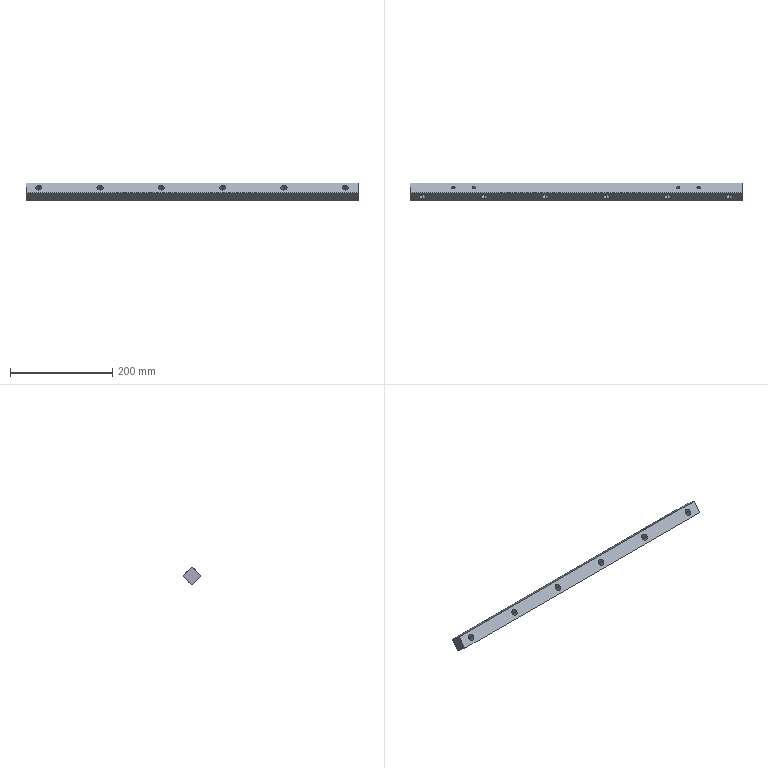Component | SolidWorks | OT-0100-001(HookSeat)-1 | 1 solid | 34 faces | box 650 x 35.17 x 35.17 mm | volume 384874 mm3 | cylinder 20 | cone 8 | plane 6 | commonest cylinder face diameters 12.5 x12 6.8 x8 | material Plain Carbon Steel
build123d program:
from build123d import *

# Parameters (mm, degrees)
SKETCH1_W             = 650
SKETCH1_H             = 25
BOSS_EXTRUDE1_DEPTH   = 25
CUT_EXTRUDE1_REACH    = 328.2
SKETCH2_R             = 6.25
M8_TAPPED_HOLE1_D     = 6.8
M8_TAPPED_HOLE1_DEPTH = 19.75
M8_TAPPED_HOLE1_TIP   = 2.043


with BuildPart() as part:
    # Sketch1 → Boss-Extrude1 (new body)
    with BuildSketch(Plane(origin=(0, 0, 0), x_dir=(1, 0, 0), z_dir=(0, 1, 0))):
        Rectangle(SKETCH1_W, SKETCH1_H)
    extrude(amount=BOSS_EXTRUDE1_DEPTH)

    # Sketch2 → Cut-Extrude1 (cut, up to next)
    with BuildSketch(Plane(origin=(0, 25, 0), x_dir=(1, 0, 0), z_dir=(0, 1, 0)), mode=Mode.PRIVATE) as cut_extrude1_sk1:
        with Locations(Location((300, 0, 0), (0, 0, 270))):
            Circle(SKETCH2_R)
    cut_extrude1_tool1 = extrude(cut_extrude1_sk1.sketch, amount=-CUT_EXTRUDE1_REACH, mode=Mode.PRIVATE) & part.part
    # Sketch2 → Cut-Extrude1 (cut, up to next)
    with BuildSketch(Plane(origin=(0, 25, 0), x_dir=(1, 0, 0), z_dir=(0, 1, 0)), mode=Mode.PRIVATE) as cut_extrude1_sk2:
        with Locations(Location((180, 0, 0), (0, 0, 270))):
            Circle(SKETCH2_R)
    cut_extrude1_tool2 = extrude(cut_extrude1_sk2.sketch, amount=-CUT_EXTRUDE1_REACH, mode=Mode.PRIVATE) & part.part
    # Sketch2 → Cut-Extrude1 (cut, up to next)
    with BuildSketch(Plane(origin=(0, 25, 0), x_dir=(1, 0, 0), z_dir=(0, 1, 0)), mode=Mode.PRIVATE) as cut_extrude1_sk3:
        with Locations(Location((60, 0, 0), (0, 0, 270))):
            Circle(SKETCH2_R)
    cut_extrude1_tool3 = extrude(cut_extrude1_sk3.sketch, amount=-CUT_EXTRUDE1_REACH, mode=Mode.PRIVATE) & part.part
    # Sketch2 → Cut-Extrude1 (cut, up to next)
    with BuildSketch(Plane(origin=(0, 25, 0), x_dir=(1, 0, 0), z_dir=(0, 1, 0)), mode=Mode.PRIVATE) as cut_extrude1_sk4:
        with Locations(Location((-60, 0, 0), (0, 0, 270))):
            Circle(SKETCH2_R)
    cut_extrude1_tool4 = extrude(cut_extrude1_sk4.sketch, amount=-CUT_EXTRUDE1_REACH, mode=Mode.PRIVATE) & part.part
    # Sketch2 → Cut-Extrude1 (cut, up to next)
    with BuildSketch(Plane(origin=(0, 25, 0), x_dir=(1, 0, 0), z_dir=(0, 1, 0)), mode=Mode.PRIVATE) as cut_extrude1_sk5:
        with Locations(Location((-180, 0, 0), (0, 0, 270))):
            Circle(SKETCH2_R)
    cut_extrude1_tool5 = extrude(cut_extrude1_sk5.sketch, amount=-CUT_EXTRUDE1_REACH, mode=Mode.PRIVATE) & part.part
    # Sketch2 → Cut-Extrude1 (cut, up to next)
    with BuildSketch(Plane(origin=(0, 25, 0), x_dir=(1, 0, 0), z_dir=(0, 1, 0)), mode=Mode.PRIVATE) as cut_extrude1_sk6:
        with Locations(Location((-300, 0, 0), (0, 0, 270))):
            Circle(SKETCH2_R)
    cut_extrude1_tool6 = extrude(cut_extrude1_sk6.sketch, amount=-CUT_EXTRUDE1_REACH, mode=Mode.PRIVATE) & part.part
    add(cut_extrude1_tool1.solids().sort_by_distance((300, 25, 0))[0], mode=Mode.SUBTRACT)
    add(cut_extrude1_tool2.solids().sort_by_distance((180, 25, 0))[0], mode=Mode.SUBTRACT)
    add(cut_extrude1_tool3.solids().sort_by_distance((60, 25, 0))[0], mode=Mode.SUBTRACT)
    add(cut_extrude1_tool4.solids().sort_by_distance((-60, 25, 0))[0], mode=Mode.SUBTRACT)
    add(cut_extrude1_tool5.solids().sort_by_distance((-180, 25, 0))[0], mode=Mode.SUBTRACT)
    add(cut_extrude1_tool6.solids().sort_by_distance((-300, 25, 0))[0], mode=Mode.SUBTRACT)

    # M8 Tapped Hole1
    with Locations(Plane.XY.offset(12.5)):
        with Locations((-240, 12.5), (240, 12.5), (-200, 12.5), (200, 12.5)):
            Hole(M8_TAPPED_HOLE1_D / 2, depth=M8_TAPPED_HOLE1_DEPTH)
            with Locations((0, 0, -(M8_TAPPED_HOLE1_DEPTH + M8_TAPPED_HOLE1_TIP / 2))):  # 118° drill point
                Cone(0, M8_TAPPED_HOLE1_D / 2, M8_TAPPED_HOLE1_TIP, mode=Mode.SUBTRACT)


solid = part.part

# Placed as in the assembly
solid = solid.moved(Location((200, -106.658, 142.812), (-39.097, 0, 0)))
STEP:
#1=COLOUR_RGB('',0.7922,0.8196,0.9333);
#2=FILL_AREA_STYLE_COLOUR('',#1);
#3=FILL_AREA_STYLE('',(#2));
#4=SURFACE_STYLE_FILL_AREA(#3);
#5=SURFACE_SIDE_STYLE('',(#4));
#6=SURFACE_STYLE_USAGE(.BOTH.,#5);
#7=PRESENTATION_STYLE_ASSIGNMENT((#6));
#8=CARTESIAN_POINT('',(-1.709,-3.997,5.091));
#9=VERTEX_POINT('',#8);
#10=CARTESIAN_POINT('',(-1.441,-3.997,5.091));
#11=VERTEX_POINT('',#10);
#12=CARTESIAN_POINT('',(-1.575,-3.997,5.091));
#13=DIRECTION('',(0.,0.6306,0.7761));
#14=DIRECTION('',(1.,0.,0.));
#15=AXIS2_PLACEMENT_3D('',#12,#13,#14);
#16=CIRCLE('',#15,0.1339);
#17=EDGE_CURVE('',#9,#11,#16,.T.);
#18=ORIENTED_EDGE('',*,*,#17,.F.);
#19=CARTESIAN_POINT('',(-1.709,-3.507,5.694));
#20=VERTEX_POINT('',#19);
#21=CARTESIAN_POINT('',(-1.709,-3.507,5.694));
#22=DIRECTION('',(0.,0.6306,0.7761));
#23=VECTOR('',#22,39.37);
#24=LINE('',#21,#23);
#25=EDGE_CURVE('',#9,#20,#24,.T.);
#26=ORIENTED_EDGE('',*,*,#25,.T.);
#27=CARTESIAN_POINT('',(-1.441,-3.507,5.694));
#28=VERTEX_POINT('',#27);
#29=CARTESIAN_POINT('',(-1.575,-3.507,5.694));
#30=DIRECTION('',(0.,0.6306,0.7761));
#31=DIRECTION('',(1.,0.,0.));
#32=AXIS2_PLACEMENT_3D('',#29,#30,#31);
#33=CIRCLE('',#32,0.1339);
#34=EDGE_CURVE('',#20,#28,#33,.T.);
#35=ORIENTED_EDGE('',*,*,#34,.T.);
#36=CARTESIAN_POINT('',(-1.441,-3.507,5.694));
#37=DIRECTION('',(0.,0.6306,0.7761));
#38=VECTOR('',#37,39.37);
#39=LINE('',#36,#38);
#40=EDGE_CURVE('',#11,#28,#39,.T.);
#41=ORIENTED_EDGE('',*,*,#40,.F.);
#42=EDGE_LOOP('',(#18,#26,#35,#41));
#43=FACE_OUTER_BOUND('',#42,.T.);
#44=CARTESIAN_POINT('',(-1.575,-3.507,5.694));
#45=DIRECTION('',(0.,0.6306,0.7761));
#46=DIRECTION('',(1.,0.,0.));
#47=AXIS2_PLACEMENT_3D('',#44,#45,#46);
#48=CYLINDRICAL_SURFACE('',#47,0.1339);
#49=ADVANCED_FACE('',(#43),#48,.F.);
#50=CARTESIAN_POINT('',(-1.575,-4.048,5.028));
#51=VERTEX_POINT('',#50);
#52=CARTESIAN_POINT('',(-1.441,-3.997,5.091));
#53=DIRECTION('',(0.8572,0.3248,0.3997));
#54=VECTOR('',#53,39.37);
#55=LINE('',#52,#54);
#56=EDGE_CURVE('',#51,#11,#55,.T.);
#57=ORIENTED_EDGE('',*,*,#56,.F.);
#58=CARTESIAN_POINT('',(-1.709,-3.997,5.091));
#59=DIRECTION('',(-0.8572,0.3248,0.3997));
#60=VECTOR('',#59,39.37);
#61=LINE('',#58,#60);
#62=EDGE_CURVE('',#51,#9,#61,.T.);
#63=ORIENTED_EDGE('',*,*,#62,.T.);
#64=ORIENTED_EDGE('',*,*,#17,.T.);
#65=EDGE_LOOP('',(#57,#63,#64));
#66=FACE_OUTER_BOUND('',#65,.T.);
#67=CARTESIAN_POINT('',(-1.575,-3.997,5.091));
#68=DIRECTION('',(0.,0.6306,0.7761));
#69=DIRECTION('',(1.,0.,0.));
#70=AXIS2_PLACEMENT_3D('',#67,#68,#69);
#71=CONICAL_SURFACE('',#70,0.1339,1.03);
#72=ADVANCED_FACE('',(#66),#71,.F.);
#73=CARTESIAN_POINT('',(17.189,-3.997,5.091));
#74=VERTEX_POINT('',#73);
#75=CARTESIAN_POINT('',(17.457,-3.997,5.091));
#76=VERTEX_POINT('',#75);
#77=CARTESIAN_POINT('',(17.323,-3.997,5.091));
#78=DIRECTION('',(0.,0.6306,0.7761));
#79=DIRECTION('',(1.,0.,0.));
#80=AXIS2_PLACEMENT_3D('',#77,#78,#79);
#81=CIRCLE('',#80,0.1339);
#82=EDGE_CURVE('',#74,#76,#81,.T.);
#83=ORIENTED_EDGE('',*,*,#82,.F.);
#84=CARTESIAN_POINT('',(17.189,-3.507,5.694));
#85=VERTEX_POINT('',#84);
#86=CARTESIAN_POINT('',(17.189,-3.507,5.694));
#87=DIRECTION('',(0.,0.6306,0.7761));
#88=VECTOR('',#87,39.37);
#89=LINE('',#86,#88);
#90=EDGE_CURVE('',#74,#85,#89,.T.);
#91=ORIENTED_EDGE('',*,*,#90,.T.);
#92=CARTESIAN_POINT('',(17.457,-3.507,5.694));
#93=VERTEX_POINT('',#92);
#94=CARTESIAN_POINT('',(17.323,-3.507,5.694));
#95=DIRECTION('',(0.,0.6306,0.7761));
#96=DIRECTION('',(1.,0.,0.));
#97=AXIS2_PLACEMENT_3D('',#94,#95,#96);
#98=CIRCLE('',#97,0.1339);
#99=EDGE_CURVE('',#85,#93,#98,.T.);
#100=ORIENTED_EDGE('',*,*,#99,.T.);
#101=CARTESIAN_POINT('',(17.457,-3.507,5.694));
#102=DIRECTION('',(0.,0.6306,0.7761));
#103=VECTOR('',#102,39.37);
#104=LINE('',#101,#103);
#105=EDGE_CURVE('',#76,#93,#104,.T.);
#106=ORIENTED_EDGE('',*,*,#105,.F.);
#107=EDGE_LOOP('',(#83,#91,#100,#106));
#108=FACE_OUTER_BOUND('',#107,.T.);
#109=CARTESIAN_POINT('',(17.323,-3.507,5.694));
#110=DIRECTION('',(0.,0.6306,0.7761));
#111=DIRECTION('',(1.,0.,0.));
#112=AXIS2_PLACEMENT_3D('',#109,#110,#111);
#113=CYLINDRICAL_SURFACE('',#112,0.1339);
#114=ADVANCED_FACE('',(#108),#113,.F.);
#115=CARTESIAN_POINT('',(17.323,-4.048,5.028));
#116=VERTEX_POINT('',#115);
#117=CARTESIAN_POINT('',(17.457,-3.997,5.091));
#118=DIRECTION('',(0.8572,0.3248,0.3997));
#119=VECTOR('',#118,39.37);
#120=LINE('',#117,#119);
#121=EDGE_CURVE('',#116,#76,#120,.T.);
#122=ORIENTED_EDGE('',*,*,#121,.F.);
#123=CARTESIAN_POINT('',(17.189,-3.997,5.091));
#124=DIRECTION('',(-0.8572,0.3248,0.3997));
#125=VECTOR('',#124,39.37);
#126=LINE('',#123,#125);
#127=EDGE_CURVE('',#116,#74,#126,.T.);
#128=ORIENTED_EDGE('',*,*,#127,.T.);
#129=ORIENTED_EDGE('',*,*,#82,.T.);
#130=EDGE_LOOP('',(#122,#128,#129));
#131=FACE_OUTER_BOUND('',#130,.T.);
#132=CARTESIAN_POINT('',(17.323,-3.997,5.091));
#133=DIRECTION('',(0.,0.6306,0.7761));
#134=DIRECTION('',(1.,0.,0.));
#135=AXIS2_PLACEMENT_3D('',#132,#133,#134);
#136=CONICAL_SURFACE('',#135,0.1339,1.03);
#137=ADVANCED_FACE('',(#131),#136,.F.);
#138=CARTESIAN_POINT('',(-0.1339,-3.997,5.091));
#139=VERTEX_POINT('',#138);
#140=CARTESIAN_POINT('',(0.1339,-3.997,5.091));
#141=VERTEX_POINT('',#140);
#142=CARTESIAN_POINT('',(0.,-3.997,5.091));
#143=DIRECTION('',(0.,0.6306,0.7761));
#144=DIRECTION('',(1.,0.,0.));
#145=AXIS2_PLACEMENT_3D('',#142,#143,#144);
#146=CIRCLE('',#145,0.1339);
#147=EDGE_CURVE('',#139,#141,#146,.T.);
#148=ORIENTED_EDGE('',*,*,#147,.F.);
#149=CARTESIAN_POINT('',(-0.1339,-3.507,5.694));
#150=VERTEX_POINT('',#149);
#151=CARTESIAN_POINT('',(-0.1339,-3.507,5.694));
#152=DIRECTION('',(0.,0.6306,0.7761));
#153=VECTOR('',#152,39.37);
#154=LINE('',#151,#153);
#155=EDGE_CURVE('',#139,#150,#154,.T.);
#156=ORIENTED_EDGE('',*,*,#155,.T.);
#157=CARTESIAN_POINT('',(0.1339,-3.507,5.694));
#158=VERTEX_POINT('',#157);
#159=CARTESIAN_POINT('',(0.,-3.507,5.694));
#160=DIRECTION('',(0.,0.6306,0.7761));
#161=DIRECTION('',(1.,0.,0.));
#162=AXIS2_PLACEMENT_3D('',#159,#160,#161);
#163=CIRCLE('',#162,0.1339);
#164=EDGE_CURVE('',#150,#158,#163,.T.);
#165=ORIENTED_EDGE('',*,*,#164,.T.);
#166=CARTESIAN_POINT('',(0.1339,-3.507,5.694));
#167=DIRECTION('',(0.,0.6306,0.7761));
#168=VECTOR('',#167,39.37);
#169=LINE('',#166,#168);
#170=EDGE_CURVE('',#141,#158,#169,.T.);
#171=ORIENTED_EDGE('',*,*,#170,.F.);
#172=EDGE_LOOP('',(#148,#156,#165,#171));
#173=FACE_OUTER_BOUND('',#172,.T.);
#174=CARTESIAN_POINT('',(0.,-3.507,5.694));
#175=DIRECTION('',(0.,0.6306,0.7761));
#176=DIRECTION('',(1.,0.,0.));
#177=AXIS2_PLACEMENT_3D('',#174,#175,#176);
#178=CYLINDRICAL_SURFACE('',#177,0.1339);
#179=ADVANCED_FACE('',(#173),#178,.F.);
#180=CARTESIAN_POINT('',(0.,-4.048,5.028));
#181=VERTEX_POINT('',#180);
#182=CARTESIAN_POINT('',(0.1339,-3.997,5.091));
#183=DIRECTION('',(0.8572,0.3248,0.3997));
#184=VECTOR('',#183,39.37);
#185=LINE('',#182,#184);
#186=EDGE_CURVE('',#181,#141,#185,.T.);
#187=ORIENTED_EDGE('',*,*,#186,.F.);
#188=CARTESIAN_POINT('',(-0.1339,-3.997,5.091));
#189=DIRECTION('',(-0.8572,0.3248,0.3997));
#190=VECTOR('',#189,39.37);
#191=LINE('',#188,#190);
#192=EDGE_CURVE('',#181,#139,#191,.T.);
#193=ORIENTED_EDGE('',*,*,#192,.T.);
#194=ORIENTED_EDGE('',*,*,#147,.T.);
#195=EDGE_LOOP('',(#187,#193,#194));
#196=FACE_OUTER_BOUND('',#195,.T.);
#197=CARTESIAN_POINT('',(0.,-3.997,5.091));
#198=DIRECTION('',(0.,0.6306,0.7761));
#199=DIRECTION('',(1.,0.,0.));
#200=AXIS2_PLACEMENT_3D('',#197,#198,#199);
#201=CONICAL_SURFACE('',#200,0.1339,1.03);
#202=ADVANCED_FACE('',(#196),#201,.F.);
#203=CARTESIAN_POINT('',(15.614,-3.997,5.091));
#204=VERTEX_POINT('',#203);
#205=CARTESIAN_POINT('',(15.882,-3.997,5.091));
#206=VERTEX_POINT('',#205);
#207=CARTESIAN_POINT('',(15.748,-3.997,5.091));
#208=DIRECTION('',(0.,0.6306,0.7761));
#209=DIRECTION('',(1.,0.,0.));
#210=AXIS2_PLACEMENT_3D('',#207,#208,#209);
#211=CIRCLE('',#210,0.1339);
#212=EDGE_CURVE('',#204,#206,#211,.T.);
#213=ORIENTED_EDGE('',*,*,#212,.F.);
#214=CARTESIAN_POINT('',(15.614,-3.507,5.694));
#215=VERTEX_POINT('',#214);
#216=CARTESIAN_POINT('',(15.614,-3.507,5.694));
#217=DIRECTION('',(0.,0.6306,0.7761));
#218=VECTOR('',#217,39.37);
#219=LINE('',#216,#218);
#220=EDGE_CURVE('',#204,#215,#219,.T.);
#221=ORIENTED_EDGE('',*,*,#220,.T.);
#222=CARTESIAN_POINT('',(15.882,-3.507,5.694));
#223=VERTEX_POINT('',#222);
#224=CARTESIAN_POINT('',(15.748,-3.507,5.694));
#225=DIRECTION('',(0.,0.6306,0.7761));
#226=DIRECTION('',(1.,0.,0.));
#227=AXIS2_PLACEMENT_3D('',#224,#225,#226);
#228=CIRCLE('',#227,0.1339);
#229=EDGE_CURVE('',#215,#223,#228,.T.);
#230=ORIENTED_EDGE('',*,*,#229,.T.);
#231=CARTESIAN_POINT('',(15.882,-3.507,5.694));
#232=DIRECTION('',(0.,0.6306,0.7761));
#233=VECTOR('',#232,39.37);
#234=LINE('',#231,#233);
#235=EDGE_CURVE('',#206,#223,#234,.T.);
#236=ORIENTED_EDGE('',*,*,#235,.F.);
#237=EDGE_LOOP('',(#213,#221,#230,#236));
#238=FACE_OUTER_BOUND('',#237,.T.);
#239=CARTESIAN_POINT('',(15.748,-3.507,5.694));
#240=DIRECTION('',(0.,0.6306,0.7761));
#241=DIRECTION('',(1.,0.,0.));
#242=AXIS2_PLACEMENT_3D('',#239,#240,#241);
#243=CYLINDRICAL_SURFACE('',#242,0.1339);
#244=ADVANCED_FACE('',(#238),#243,.F.);
#245=CARTESIAN_POINT('',(15.748,-4.048,5.028));
#246=VERTEX_POINT('',#245);
#247=CARTESIAN_POINT('',(15.882,-3.997,5.091));
#248=DIRECTION('',(0.8572,0.3248,0.3997));
#249=VECTOR('',#248,39.37);
#250=LINE('',#247,#249);
#251=EDGE_CURVE('',#246,#206,#250,.T.);
#252=ORIENTED_EDGE('',*,*,#251,.F.);
#253=CARTESIAN_POINT('',(15.614,-3.997,5.091));
#254=DIRECTION('',(-0.8572,0.3248,0.3997));
#255=VECTOR('',#254,39.37);
#256=LINE('',#253,#255);
#257=EDGE_CURVE('',#246,#204,#256,.T.);
#258=ORIENTED_EDGE('',*,*,#257,.T.);
#259=ORIENTED_EDGE('',*,*,#212,.T.);
#260=EDGE_LOOP('',(#252,#258,#259));
#261=FACE_OUTER_BOUND('',#260,.T.);
#262=CARTESIAN_POINT('',(15.748,-3.997,5.091));
#263=DIRECTION('',(0.,0.6306,0.7761));
#264=DIRECTION('',(1.,0.,0.));
#265=AXIS2_PLACEMENT_3D('',#262,#263,#264);
#266=CONICAL_SURFACE('',#265,0.1339,1.03);
#267=ADVANCED_FACE('',(#261),#266,.F.);
#268=CARTESIAN_POINT('',(-3.937,-4.354,5.432));
#269=VERTEX_POINT('',#268);
#270=CARTESIAN_POINT('',(-3.937,-4.044,5.813));
#271=VERTEX_POINT('',#270);
#272=CARTESIAN_POINT('',(-3.937,-4.199,5.623));
#273=DIRECTION('',(-0.,0.7761,-0.6306));
#274=DIRECTION('',(0.,-0.6306,-0.7761));
#275=AXIS2_PLACEMENT_3D('',#272,#273,#274);
#276=CIRCLE('',#275,0.2461);
#277=EDGE_CURVE('',#269,#271,#276,.T.);
#278=ORIENTED_EDGE('',*,*,#277,.F.);
#279=CARTESIAN_POINT('',(-3.937,-3.59,4.811));
#280=VERTEX_POINT('',#279);
#281=CARTESIAN_POINT('',(-3.937,-4.354,5.432));
#282=DIRECTION('',(-0.,0.7761,-0.6306));
#283=VECTOR('',#282,39.37);
#284=LINE('',#281,#283);
#285=EDGE_CURVE('',#269,#280,#284,.T.);
#286=ORIENTED_EDGE('',*,*,#285,.T.);
#287=CARTESIAN_POINT('',(-3.937,-3.28,5.193));
#288=VERTEX_POINT('',#287);
#289=CARTESIAN_POINT('',(-3.937,-3.435,5.002));
#290=DIRECTION('',(-0.,0.7761,-0.6306));
#291=DIRECTION('',(0.,0.6306,0.7761));
#292=AXIS2_PLACEMENT_3D('',#289,#290,#291);
#293=CIRCLE('',#292,0.2461);
#294=EDGE_CURVE('',#280,#288,#293,.T.);
#295=ORIENTED_EDGE('',*,*,#294,.T.);
#296=CARTESIAN_POINT('',(-3.937,-4.044,5.814));
#297=DIRECTION('',(-0.,0.7761,-0.6306));
#298=VECTOR('',#297,39.37);
#299=LINE('',#296,#298);
#300=EDGE_CURVE('',#271,#288,#299,.T.);
#301=ORIENTED_EDGE('',*,*,#300,.F.);
#302=EDGE_LOOP('',(#278,#286,#295,#301));
#303=FACE_OUTER_BOUND('',#302,.T.);
#304=CARTESIAN_POINT('',(-3.937,-4.199,5.623));
#305=DIRECTION('',(-0.,0.7761,-0.6306));
#306=DIRECTION('',(0.,0.6306,0.7761));
#307=AXIS2_PLACEMENT_3D('',#304,#305,#306);
#308=CYLINDRICAL_SURFACE('',#307,0.2461);
#309=ADVANCED_FACE('',(#303),#308,.F.);
#310=CARTESIAN_POINT('',(0.7874,-4.354,5.432));
#311=VERTEX_POINT('',#310);
#312=CARTESIAN_POINT('',(0.7874,-4.044,5.813));
#313=VERTEX_POINT('',#312);
#314=CARTESIAN_POINT('',(0.7874,-4.199,5.623));
#315=DIRECTION('',(-0.,0.7761,-0.6306));
#316=DIRECTION('',(0.,-0.6306,-0.7761));
#317=AXIS2_PLACEMENT_3D('',#314,#315,#316);
#318=CIRCLE('',#317,0.2461);
#319=EDGE_CURVE('',#311,#313,#318,.T.);
#320=ORIENTED_EDGE('',*,*,#319,.F.);
#321=CARTESIAN_POINT('',(0.7874,-3.59,4.811));
#322=VERTEX_POINT('',#321);
#323=CARTESIAN_POINT('',(0.7874,-4.354,5.432));
#324=DIRECTION('',(-0.,0.7761,-0.6306));
#325=VECTOR('',#324,39.37);
#326=LINE('',#323,#325);
#327=EDGE_CURVE('',#311,#322,#326,.T.);
#328=ORIENTED_EDGE('',*,*,#327,.T.);
#329=CARTESIAN_POINT('',(0.7874,-3.28,5.193));
#330=VERTEX_POINT('',#329);
#331=CARTESIAN_POINT('',(0.7874,-3.435,5.002));
#332=DIRECTION('',(-0.,0.7761,-0.6306));
#333=DIRECTION('',(0.,0.6306,0.7761));
#334=AXIS2_PLACEMENT_3D('',#331,#332,#333);
#335=CIRCLE('',#334,0.2461);
#336=EDGE_CURVE('',#322,#330,#335,.T.);
#337=ORIENTED_EDGE('',*,*,#336,.T.);
#338=CARTESIAN_POINT('',(0.7874,-4.044,5.814));
#339=DIRECTION('',(-0.,0.7761,-0.6306));
#340=VECTOR('',#339,39.37);
#341=LINE('',#338,#340);
#342=EDGE_CURVE('',#313,#330,#341,.T.);
#343=ORIENTED_EDGE('',*,*,#342,.F.);
#344=EDGE_LOOP('',(#320,#328,#337,#343));
#345=FACE_OUTER_BOUND('',#344,.T.);
#346=CARTESIAN_POINT('',(0.7874,-4.199,5.623));
#347=DIRECTION('',(-0.,0.7761,-0.6306));
#348=DIRECTION('',(0.,0.6306,0.7761));
#349=AXIS2_PLACEMENT_3D('',#346,#347,#348);
#350=CYLINDRICAL_SURFACE('',#349,0.2461);
#351=ADVANCED_FACE('',(#345),#350,.F.);
#352=CARTESIAN_POINT('',(5.512,-4.354,5.432));
#353=VERTEX_POINT('',#352);
#354=CARTESIAN_POINT('',(5.512,-4.044,5.813));
#355=VERTEX_POINT('',#354);
#356=CARTESIAN_POINT('',(5.512,-4.199,5.623));
#357=DIRECTION('',(-0.,0.7761,-0.6306));
#358=DIRECTION('',(0.,-0.6306,-0.7761));
#359=AXIS2_PLACEMENT_3D('',#356,#357,#358);
#360=CIRCLE('',#359,0.2461);
#361=EDGE_CURVE('',#353,#355,#360,.T.);
#362=ORIENTED_EDGE('',*,*,#361,.F.);
#363=CARTESIAN_POINT('',(5.512,-3.59,4.811));
#364=VERTEX_POINT('',#363);
#365=CARTESIAN_POINT('',(5.512,-4.354,5.432));
#366=DIRECTION('',(-0.,0.7761,-0.6306));
#367=VECTOR('',#366,39.37);
#368=LINE('',#365,#367);
#369=EDGE_CURVE('',#353,#364,#368,.T.);
#370=ORIENTED_EDGE('',*,*,#369,.T.);
#371=CARTESIAN_POINT('',(5.512,-3.28,5.193));
#372=VERTEX_POINT('',#371);
#373=CARTESIAN_POINT('',(5.512,-3.435,5.002));
#374=DIRECTION('',(-0.,0.7761,-0.6306));
#375=DIRECTION('',(0.,0.6306,0.7761));
#376=AXIS2_PLACEMENT_3D('',#373,#374,#375);
#377=CIRCLE('',#376,0.2461);
#378=EDGE_CURVE('',#364,#372,#377,.T.);
#379=ORIENTED_EDGE('',*,*,#378,.T.);
#380=CARTESIAN_POINT('',(5.512,-4.044,5.814));
#381=DIRECTION('',(-0.,0.7761,-0.6306));
#382=VECTOR('',#381,39.37);
#383=LINE('',#380,#382);
#384=EDGE_CURVE('',#355,#372,#383,.T.);
#385=ORIENTED_EDGE('',*,*,#384,.F.);
#386=EDGE_LOOP('',(#362,#370,#379,#385));
#387=FACE_OUTER_BOUND('',#386,.T.);
#388=CARTESIAN_POINT('',(5.512,-4.199,5.623));
#389=DIRECTION('',(-0.,0.7761,-0.6306));
#390=DIRECTION('',(0.,0.6306,0.7761));
#391=AXIS2_PLACEMENT_3D('',#388,#389,#390);
#392=CYLINDRICAL_SURFACE('',#391,0.2461);
#393=ADVANCED_FACE('',(#387),#392,.F.);
#394=CARTESIAN_POINT('',(10.236,-4.354,5.432));
#395=VERTEX_POINT('',#394);
#396=CARTESIAN_POINT('',(10.236,-4.044,5.813));
#397=VERTEX_POINT('',#396);
#398=CARTESIAN_POINT('',(10.236,-4.199,5.623));
#399=DIRECTION('',(-0.,0.7761,-0.6306));
#400=DIRECTION('',(0.,-0.6306,-0.7761));
#401=AXIS2_PLACEMENT_3D('',#398,#399,#400);
#402=CIRCLE('',#401,0.2461);
#403=EDGE_CURVE('',#395,#397,#402,.T.);
#404=ORIENTED_EDGE('',*,*,#403,.F.);
#405=CARTESIAN_POINT('',(10.236,-3.59,4.811));
#406=VERTEX_POINT('',#405);
#407=CARTESIAN_POINT('',(10.236,-4.354,5.432));
#408=DIRECTION('',(-0.,0.7761,-0.6306));
#409=VECTOR('',#408,39.37);
#410=LINE('',#407,#409);
#411=EDGE_CURVE('',#395,#406,#410,.T.);
#412=ORIENTED_EDGE('',*,*,#411,.T.);
#413=CARTESIAN_POINT('',(10.236,-3.28,5.193));
#414=VERTEX_POINT('',#413);
#415=CARTESIAN_POINT('',(10.236,-3.435,5.002));
#416=DIRECTION('',(-0.,0.7761,-0.6306));
#417=DIRECTION('',(0.,0.6306,0.7761));
#418=AXIS2_PLACEMENT_3D('',#415,#416,#417);
#419=CIRCLE('',#418,0.2461);
#420=EDGE_CURVE('',#406,#414,#419,.T.);
#421=ORIENTED_EDGE('',*,*,#420,.T.);
#422=CARTESIAN_POINT('',(10.236,-4.044,5.814));
#423=DIRECTION('',(-0.,0.7761,-0.6306));
#424=VECTOR('',#423,39.37);
#425=LINE('',#422,#424);
#426=EDGE_CURVE('',#397,#414,#425,.T.);
#427=ORIENTED_EDGE('',*,*,#426,.F.);
#428=EDGE_LOOP('',(#404,#412,#421,#427));
#429=FACE_OUTER_BOUND('',#428,.T.);
#430=CARTESIAN_POINT('',(10.236,-4.199,5.623));
#431=DIRECTION('',(-0.,0.7761,-0.6306));
#432=DIRECTION('',(0.,0.6306,0.7761));
#433=AXIS2_PLACEMENT_3D('',#430,#431,#432);
#434=CYLINDRICAL_SURFACE('',#433,0.2461);
#435=ADVANCED_FACE('',(#429),#434,.F.);
#436=CARTESIAN_POINT('',(14.961,-4.354,5.432));
#437=VERTEX_POINT('',#436);
#438=CARTESIAN_POINT('',(14.961,-4.044,5.813));
#439=VERTEX_POINT('',#438);
#440=CARTESIAN_POINT('',(14.961,-4.199,5.623));
#441=DIRECTION('',(-0.,0.7761,-0.6306));
#442=DIRECTION('',(0.,-0.6306,-0.7761));
#443=AXIS2_PLACEMENT_3D('',#440,#441,#442);
#444=CIRCLE('',#443,0.2461);
#445=EDGE_CURVE('',#437,#439,#444,.T.);
#446=ORIENTED_EDGE('',*,*,#445,.F.);
#447=CARTESIAN_POINT('',(14.961,-3.59,4.811));
#448=VERTEX_POINT('',#447);
#449=CARTESIAN_POINT('',(14.961,-4.354,5.432));
#450=DIRECTION('',(-0.,0.7761,-0.6306));
#451=VECTOR('',#450,39.37);
#452=LINE('',#449,#451);
#453=EDGE_CURVE('',#437,#448,#452,.T.);
#454=ORIENTED_EDGE('',*,*,#453,.T.);
#455=CARTESIAN_POINT('',(14.961,-3.28,5.193));
#456=VERTEX_POINT('',#455);
#457=CARTESIAN_POINT('',(14.961,-3.435,5.002));
#458=DIRECTION('',(-0.,0.7761,-0.6306));
#459=DIRECTION('',(0.,0.6306,0.7761));
#460=AXIS2_PLACEMENT_3D('',#457,#458,#459);
#461=CIRCLE('',#460,0.2461);
#462=EDGE_CURVE('',#448,#456,#461,.T.);
#463=ORIENTED_EDGE('',*,*,#462,.T.);
#464=CARTESIAN_POINT('',(14.961,-4.044,5.814));
#465=DIRECTION('',(-0.,0.7761,-0.6306));
#466=VECTOR('',#465,39.37);
#467=LINE('',#464,#466);
#468=EDGE_CURVE('',#439,#456,#467,.T.);
#469=ORIENTED_EDGE('',*,*,#468,.F.);
#470=EDGE_LOOP('',(#446,#454,#463,#469));
#471=FACE_OUTER_BOUND('',#470,.T.);
#472=CARTESIAN_POINT('',(14.961,-4.199,5.623));
#473=DIRECTION('',(-0.,0.7761,-0.6306));
#474=DIRECTION('',(0.,0.6306,0.7761));
#475=AXIS2_PLACEMENT_3D('',#472,#473,#474);
#476=CYLINDRICAL_SURFACE('',#475,0.2461);
#477=ADVANCED_FACE('',(#471),#476,.F.);
#478=CARTESIAN_POINT('',(19.685,-4.354,5.432));
#479=VERTEX_POINT('',#478);
#480=CARTESIAN_POINT('',(19.685,-4.044,5.813));
#481=VERTEX_POINT('',#480);
#482=CARTESIAN_POINT('',(19.685,-4.199,5.623));
#483=DIRECTION('',(-0.,0.7761,-0.6306));
#484=DIRECTION('',(0.,-0.6306,-0.7761));
#485=AXIS2_PLACEMENT_3D('',#482,#483,#484);
#486=CIRCLE('',#485,0.2461);
#487=EDGE_CURVE('',#479,#481,#486,.T.);
#488=ORIENTED_EDGE('',*,*,#487,.F.);
#489=CARTESIAN_POINT('',(19.685,-3.59,4.811));
#490=VERTEX_POINT('',#489);
#491=CARTESIAN_POINT('',(19.685,-4.354,5.432));
#492=DIRECTION('',(-0.,0.7761,-0.6306));
#493=VECTOR('',#492,39.37);
#494=LINE('',#491,#493);
#495=EDGE_CURVE('',#479,#490,#494,.T.);
#496=ORIENTED_EDGE('',*,*,#495,.T.);
#497=CARTESIAN_POINT('',(19.685,-3.28,5.193));
#498=VERTEX_POINT('',#497);
#499=CARTESIAN_POINT('',(19.685,-3.435,5.002));
#500=DIRECTION('',(-0.,0.7761,-0.6306));
#501=DIRECTION('',(0.,0.6306,0.7761));
#502=AXIS2_PLACEMENT_3D('',#499,#500,#501);
#503=CIRCLE('',#502,0.2461);
#504=EDGE_CURVE('',#490,#498,#503,.T.);
#505=ORIENTED_EDGE('',*,*,#504,.T.);
#506=CARTESIAN_POINT('',(19.685,-4.044,5.814));
#507=DIRECTION('',(-0.,0.7761,-0.6306));
#508=VECTOR('',#507,39.37);
#509=LINE('',#506,#508);
#510=EDGE_CURVE('',#481,#498,#509,.T.);
#511=ORIENTED_EDGE('',*,*,#510,.F.);
#512=EDGE_LOOP('',(#488,#496,#505,#511));
#513=FACE_OUTER_BOUND('',#512,.T.);
#514=CARTESIAN_POINT('',(19.685,-4.199,5.623));
#515=DIRECTION('',(-0.,0.7761,-0.6306));
#516=DIRECTION('',(0.,0.6306,0.7761));
#517=AXIS2_PLACEMENT_3D('',#514,#515,#516);
#518=CYLINDRICAL_SURFACE('',#517,0.2461);
#519=ADVANCED_FACE('',(#513),#518,.F.);
#520=CARTESIAN_POINT('',(20.669,-3.889,6.004));
#521=VERTEX_POINT('',#520);
#522=CARTESIAN_POINT('',(20.669,-4.509,5.241));
#523=VERTEX_POINT('',#522);
#524=CARTESIAN_POINT('',(20.669,-3.889,6.004));
#525=DIRECTION('',(-0.,-0.6306,-0.7761));
#526=VECTOR('',#525,39.37);
#527=LINE('',#524,#526);
#528=EDGE_CURVE('',#521,#523,#527,.T.);
#529=ORIENTED_EDGE('',*,*,#528,.T.);
#530=CARTESIAN_POINT('',(20.669,-3.746,4.62));
#531=VERTEX_POINT('',#530);
#532=CARTESIAN_POINT('',(20.669,-3.746,4.62));
#533=DIRECTION('',(0.,-0.7761,0.6306));
#534=VECTOR('',#533,39.37);
#535=LINE('',#532,#534);
#536=EDGE_CURVE('',#531,#523,#535,.T.);
#537=ORIENTED_EDGE('',*,*,#536,.F.);
#538=CARTESIAN_POINT('',(20.669,-3.125,5.384));
#539=VERTEX_POINT('',#538);
#540=CARTESIAN_POINT('',(20.669,-3.125,5.384));
#541=DIRECTION('',(-0.,-0.6306,-0.7761));
#542=VECTOR('',#541,39.37);
#543=LINE('',#540,#542);
#544=EDGE_CURVE('',#539,#531,#543,.T.);
#545=ORIENTED_EDGE('',*,*,#544,.F.);
#546=CARTESIAN_POINT('',(20.669,-3.125,5.384));
#547=DIRECTION('',(0.,-0.7761,0.6306));
#548=VECTOR('',#547,39.37);
#549=LINE('',#546,#548);
#550=EDGE_CURVE('',#539,#521,#549,.T.);
#551=ORIENTED_EDGE('',*,*,#550,.T.);
#552=EDGE_LOOP('',(#529,#537,#545,#551));
#553=FACE_OUTER_BOUND('',#552,.T.);
#554=CARTESIAN_POINT('',(20.669,-3.125,5.384));
#555=DIRECTION('',(-1.,-0.,0.));
#556=DIRECTION('',(0.,0.6306,0.7761));
#557=AXIS2_PLACEMENT_3D('',#554,#555,#556);
#558=PLANE('',#557);
#559=ADVANCED_FACE('',(#553),#558,.F.);
#560=CARTESIAN_POINT('',(-4.921,-4.509,5.241));
#561=VERTEX_POINT('',#560);
#562=CARTESIAN_POINT('',(-4.921,-4.509,5.241));
#563=DIRECTION('',(-1.,-0.,0.));
#564=VECTOR('',#563,39.37);
#565=LINE('',#562,#564);
#566=EDGE_CURVE('',#523,#561,#565,.T.);
#567=ORIENTED_EDGE('',*,*,#566,.T.);
#568=CARTESIAN_POINT('',(-4.921,-3.746,4.62));
#569=VERTEX_POINT('',#568);
#570=CARTESIAN_POINT('',(-4.921,-3.746,4.62));
#571=DIRECTION('',(0.,-0.7761,0.6306));
#572=VECTOR('',#571,39.37);
#573=LINE('',#570,#572);
#574=EDGE_CURVE('',#569,#561,#573,.T.);
#575=ORIENTED_EDGE('',*,*,#574,.F.);
#576=CARTESIAN_POINT('',(-4.921,-3.746,4.62));
#577=DIRECTION('',(-1.,-0.,0.));
#578=VECTOR('',#577,39.37);
#579=LINE('',#576,#578);
#580=EDGE_CURVE('',#531,#569,#579,.T.);
#581=ORIENTED_EDGE('',*,*,#580,.F.);
#582=ORIENTED_EDGE('',*,*,#536,.T.);
#583=EDGE_LOOP('',(#567,#575,#581,#582));
#584=FACE_OUTER_BOUND('',#583,.T.);
#585=CARTESIAN_POINT('',(-4.921,-3.746,4.62));
#586=DIRECTION('',(0.,0.6306,0.7761));
#587=DIRECTION('',(1.,0.,-0.));
#588=AXIS2_PLACEMENT_3D('',#585,#586,#587);
#589=PLANE('',#588);
#590=ADVANCED_FACE('',(#584),#589,.F.);
#591=CARTESIAN_POINT('',(-4.921,-3.889,6.004));
#592=VERTEX_POINT('',#591);
#593=CARTESIAN_POINT('',(-4.921,-3.889,6.004));
#594=DIRECTION('',(0.,0.6306,0.7761));
#595=VECTOR('',#594,39.37);
#596=LINE('',#593,#595);
#597=EDGE_CURVE('',#561,#592,#596,.T.);
#598=ORIENTED_EDGE('',*,*,#597,.T.);
#599=CARTESIAN_POINT('',(-4.921,-3.125,5.384));
#600=VERTEX_POINT('',#599);
#601=CARTESIAN_POINT('',(-4.921,-3.125,5.384));
#602=DIRECTION('',(0.,-0.7761,0.6306));
#603=VECTOR('',#602,39.37);
#604=LINE('',#601,#603);
#605=EDGE_CURVE('',#600,#592,#604,.T.);
#606=ORIENTED_EDGE('',*,*,#605,.F.);
#607=CARTESIAN_POINT('',(-4.921,-3.125,5.384));
#608=DIRECTION('',(0.,0.6306,0.7761));
#609=VECTOR('',#608,39.37);
#610=LINE('',#607,#609);
#611=EDGE_CURVE('',#569,#600,#610,.T.);
#612=ORIENTED_EDGE('',*,*,#611,.F.);
#613=ORIENTED_EDGE('',*,*,#574,.T.);
#614=EDGE_LOOP('',(#598,#606,#612,#613));
#615=FACE_OUTER_BOUND('',#614,.T.);
#616=CARTESIAN_POINT('',(-4.921,-3.125,5.384));
#617=DIRECTION('',(1.,0.,-0.));
#618=DIRECTION('',(-0.,-0.6306,-0.7761));
#619=AXIS2_PLACEMENT_3D('',#616,#617,#618);
#620=PLANE('',#619);
#621=ADVANCED_FACE('',(#615),#620,.F.);
#622=CARTESIAN_POINT('',(-1.575,-3.507,5.694));
#623=DIRECTION('',(0.,0.6306,0.7761));
#624=DIRECTION('',(1.,0.,0.));
#625=AXIS2_PLACEMENT_3D('',#622,#623,#624);
#626=CIRCLE('',#625,0.1339);
#627=EDGE_CURVE('',#28,#20,#626,.T.);
#628=ORIENTED_EDGE('',*,*,#627,.F.);
#629=ORIENTED_EDGE('',*,*,#34,.F.);
#630=EDGE_LOOP('',(#628,#629));
#631=FACE_BOUND('',#630,.T.);
#632=CARTESIAN_POINT('',(17.323,-3.507,5.694));
#633=DIRECTION('',(0.,0.6306,0.7761));
#634=DIRECTION('',(1.,0.,0.));
#635=AXIS2_PLACEMENT_3D('',#632,#633,#634);
#636=CIRCLE('',#635,0.1339);
#637=EDGE_CURVE('',#93,#85,#636,.T.);
#638=ORIENTED_EDGE('',*,*,#637,.F.);
#639=ORIENTED_EDGE('',*,*,#99,.F.);
#640=EDGE_LOOP('',(#638,#639));
#641=FACE_BOUND('',#640,.T.);
#642=CARTESIAN_POINT('',(0.,-3.507,5.694));
#643=DIRECTION('',(0.,0.6306,0.7761));
#644=DIRECTION('',(1.,0.,0.));
#645=AXIS2_PLACEMENT_3D('',#642,#643,#644);
#646=CIRCLE('',#645,0.1339);
#647=EDGE_CURVE('',#158,#150,#646,.T.);
#648=ORIENTED_EDGE('',*,*,#647,.F.);
#649=ORIENTED_EDGE('',*,*,#164,.F.);
#650=EDGE_LOOP('',(#648,#649));
#651=FACE_BOUND('',#650,.T.);
#652=CARTESIAN_POINT('',(15.748,-3.507,5.694));
#653=DIRECTION('',(0.,0.6306,0.7761));
#654=DIRECTION('',(1.,0.,0.));
#655=AXIS2_PLACEMENT_3D('',#652,#653,#654);
#656=CIRCLE('',#655,0.1339);
#657=EDGE_CURVE('',#223,#215,#656,.T.);
#658=ORIENTED_EDGE('',*,*,#657,.F.);
#659=ORIENTED_EDGE('',*,*,#229,.F.);
#660=EDGE_LOOP('',(#658,#659));
#661=FACE_BOUND('',#660,.T.);
#662=CARTESIAN_POINT('',(-4.921,-3.889,6.004));
#663=DIRECTION('',(1.,0.,-0.));
#664=VECTOR('',#663,39.37);
#665=LINE('',#662,#664);
#666=EDGE_CURVE('',#592,#521,#665,.T.);
#667=ORIENTED_EDGE('',*,*,#666,.T.);
#668=ORIENTED_EDGE('',*,*,#550,.F.);
#669=CARTESIAN_POINT('',(-4.921,-3.125,5.384));
#670=DIRECTION('',(1.,0.,-0.));
#671=VECTOR('',#670,39.37);
#672=LINE('',#669,#671);
#673=EDGE_CURVE('',#600,#539,#672,.T.);
#674=ORIENTED_EDGE('',*,*,#673,.F.);
#675=ORIENTED_EDGE('',*,*,#605,.T.);
#676=EDGE_LOOP('',(#667,#668,#674,#675));
#677=FACE_OUTER_BOUND('',#676,.T.);
#678=CARTESIAN_POINT('',(-4.921,-3.125,5.384));
#679=DIRECTION('',(-0.,-0.6306,-0.7761));
#680=DIRECTION('',(-1.,-0.,0.));
#681=AXIS2_PLACEMENT_3D('',#678,#679,#680);
#682=PLANE('',#681);
#683=ADVANCED_FACE('',(#631,#641,#651,#661,#677),#682,.F.);
#684=CARTESIAN_POINT('',(-3.937,-3.435,5.002));
#685=DIRECTION('',(-0.,0.7761,-0.6306));
#686=DIRECTION('',(0.,0.6306,0.7761));
#687=AXIS2_PLACEMENT_3D('',#684,#685,#686);
#688=CIRCLE('',#687,0.2461);
#689=EDGE_CURVE('',#288,#280,#688,.T.);
#690=ORIENTED_EDGE('',*,*,#689,.F.);
#691=ORIENTED_EDGE('',*,*,#294,.F.);
#692=EDGE_LOOP('',(#690,#691));
#693=FACE_BOUND('',#692,.T.);
#694=CARTESIAN_POINT('',(0.7874,-3.435,5.002));
#695=DIRECTION('',(-0.,0.7761,-0.6306));
#696=DIRECTION('',(0.,0.6306,0.7761));
#697=AXIS2_PLACEMENT_3D('',#694,#695,#696);
#698=CIRCLE('',#697,0.2461);
#699=EDGE_CURVE('',#330,#322,#698,.T.);
#700=ORIENTED_EDGE('',*,*,#699,.F.);
#701=ORIENTED_EDGE('',*,*,#336,.F.);
#702=EDGE_LOOP('',(#700,#701));
#703=FACE_BOUND('',#702,.T.);
#704=CARTESIAN_POINT('',(5.512,-3.435,5.002));
#705=DIRECTION('',(-0.,0.7761,-0.6306));
#706=DIRECTION('',(0.,0.6306,0.7761));
#707=AXIS2_PLACEMENT_3D('',#704,#705,#706);
#708=CIRCLE('',#707,0.2461);
#709=EDGE_CURVE('',#372,#364,#708,.T.);
#710=ORIENTED_EDGE('',*,*,#709,.F.);
#711=ORIENTED_EDGE('',*,*,#378,.F.);
#712=EDGE_LOOP('',(#710,#711));
#713=FACE_BOUND('',#712,.T.);
#714=CARTESIAN_POINT('',(10.236,-3.435,5.002));
#715=DIRECTION('',(-0.,0.7761,-0.6306));
#716=DIRECTION('',(0.,0.6306,0.7761));
#717=AXIS2_PLACEMENT_3D('',#714,#715,#716);
#718=CIRCLE('',#717,0.2461);
#719=EDGE_CURVE('',#414,#406,#718,.T.);
#720=ORIENTED_EDGE('',*,*,#719,.F.);
#721=ORIENTED_EDGE('',*,*,#420,.F.);
#722=EDGE_LOOP('',(#720,#721));
#723=FACE_BOUND('',#722,.T.);
#724=CARTESIAN_POINT('',(14.961,-3.435,5.002));
#725=DIRECTION('',(-0.,0.7761,-0.6306));
#726=DIRECTION('',(0.,0.6306,0.7761));
#727=AXIS2_PLACEMENT_3D('',#724,#725,#726);
#728=CIRCLE('',#727,0.2461);
#729=EDGE_CURVE('',#456,#448,#728,.T.);
#730=ORIENTED_EDGE('',*,*,#729,.F.);
#731=ORIENTED_EDGE('',*,*,#462,.F.);
#732=EDGE_LOOP('',(#730,#731));
#733=FACE_BOUND('',#732,.T.);
#734=CARTESIAN_POINT('',(19.685,-3.435,5.002));
#735=DIRECTION('',(-0.,0.7761,-0.6306));
#736=DIRECTION('',(0.,0.6306,0.7761));
#737=AXIS2_PLACEMENT_3D('',#734,#735,#736);
#738=CIRCLE('',#737,0.2461);
#739=EDGE_CURVE('',#498,#490,#738,.T.);
#740=ORIENTED_EDGE('',*,*,#739,.F.);
#741=ORIENTED_EDGE('',*,*,#504,.F.);
#742=EDGE_LOOP('',(#740,#741));
#743=FACE_BOUND('',#742,.T.);
#744=ORIENTED_EDGE('',*,*,#544,.T.);
#745=ORIENTED_EDGE('',*,*,#580,.T.);
#746=ORIENTED_EDGE('',*,*,#611,.T.);
#747=ORIENTED_EDGE('',*,*,#673,.T.);
#748=EDGE_LOOP('',(#744,#745,#746,#747));
#749=FACE_OUTER_BOUND('',#748,.T.);
#750=CARTESIAN_POINT('',(7.874,-3.435,5.002));
#751=DIRECTION('',(0.,-0.7761,0.6306));
#752=DIRECTION('',(-0.,-0.6306,-0.7761));
#753=AXIS2_PLACEMENT_3D('',#750,#751,#752);
#754=PLANE('',#753);
#755=ADVANCED_FACE('',(#693,#703,#713,#723,#733,#743,#749),#754,.F.);
#756=CARTESIAN_POINT('',(-3.937,-4.199,5.623));
#757=DIRECTION('',(-0.,0.7761,-0.6306));
#758=DIRECTION('',(0.,-0.6306,-0.7761));
#759=AXIS2_PLACEMENT_3D('',#756,#757,#758);
#760=CIRCLE('',#759,0.2461);
#761=EDGE_CURVE('',#271,#269,#760,.T.);
#762=ORIENTED_EDGE('',*,*,#761,.T.);
#763=ORIENTED_EDGE('',*,*,#277,.T.);
#764=EDGE_LOOP('',(#762,#763));
#765=FACE_BOUND('',#764,.T.);
#766=CARTESIAN_POINT('',(0.7874,-4.199,5.623));
#767=DIRECTION('',(-0.,0.7761,-0.6306));
#768=DIRECTION('',(0.,-0.6306,-0.7761));
#769=AXIS2_PLACEMENT_3D('',#766,#767,#768);
#770=CIRCLE('',#769,0.2461);
#771=EDGE_CURVE('',#313,#311,#770,.T.);
#772=ORIENTED_EDGE('',*,*,#771,.T.);
#773=ORIENTED_EDGE('',*,*,#319,.T.);
#774=EDGE_LOOP('',(#772,#773));
#775=FACE_BOUND('',#774,.T.);
#776=CARTESIAN_POINT('',(5.512,-4.199,5.623));
#777=DIRECTION('',(-0.,0.7761,-0.6306));
#778=DIRECTION('',(0.,-0.6306,-0.7761));
#779=AXIS2_PLACEMENT_3D('',#776,#777,#778);
#780=CIRCLE('',#779,0.2461);
#781=EDGE_CURVE('',#355,#353,#780,.T.);
#782=ORIENTED_EDGE('',*,*,#781,.T.);
#783=ORIENTED_EDGE('',*,*,#361,.T.);
#784=EDGE_LOOP('',(#782,#783));
#785=FACE_BOUND('',#784,.T.);
#786=CARTESIAN_POINT('',(10.236,-4.199,5.623));
#787=DIRECTION('',(-0.,0.7761,-0.6306));
#788=DIRECTION('',(0.,-0.6306,-0.7761));
#789=AXIS2_PLACEMENT_3D('',#786,#787,#788);
#790=CIRCLE('',#789,0.2461);
#791=EDGE_CURVE('',#397,#395,#790,.T.);
#792=ORIENTED_EDGE('',*,*,#791,.T.);
#793=ORIENTED_EDGE('',*,*,#403,.T.);
#794=EDGE_LOOP('',(#792,#793));
#795=FACE_BOUND('',#794,.T.);
#796=CARTESIAN_POINT('',(14.961,-4.199,5.623));
#797=DIRECTION('',(-0.,0.7761,-0.6306));
#798=DIRECTION('',(0.,-0.6306,-0.7761));
#799=AXIS2_PLACEMENT_3D('',#796,#797,#798);
#800=CIRCLE('',#799,0.2461);
#801=EDGE_CURVE('',#439,#437,#800,.T.);
#802=ORIENTED_EDGE('',*,*,#801,.T.);
#803=ORIENTED_EDGE('',*,*,#445,.T.);
#804=EDGE_LOOP('',(#802,#803));
#805=FACE_BOUND('',#804,.T.);
#806=CARTESIAN_POINT('',(19.685,-4.199,5.623));
#807=DIRECTION('',(-0.,0.7761,-0.6306));
#808=DIRECTION('',(0.,-0.6306,-0.7761));
#809=AXIS2_PLACEMENT_3D('',#806,#807,#808);
#810=CIRCLE('',#809,0.2461);
#811=EDGE_CURVE('',#481,#479,#810,.T.);
#812=ORIENTED_EDGE('',*,*,#811,.T.);
#813=ORIENTED_EDGE('',*,*,#487,.T.);
#814=EDGE_LOOP('',(#812,#813));
#815=FACE_BOUND('',#814,.T.);
#816=ORIENTED_EDGE('',*,*,#528,.F.);
#817=ORIENTED_EDGE('',*,*,#666,.F.);
#818=ORIENTED_EDGE('',*,*,#597,.F.);
#819=ORIENTED_EDGE('',*,*,#566,.F.);
#820=EDGE_LOOP('',(#816,#817,#818,#819));
#821=FACE_OUTER_BOUND('',#820,.T.);
#822=CARTESIAN_POINT('',(7.874,-4.199,5.623));
#823=DIRECTION('',(0.,-0.7761,0.6306));
#824=DIRECTION('',(-0.,-0.6306,-0.7761));
#825=AXIS2_PLACEMENT_3D('',#822,#823,#824);
#826=PLANE('',#825);
#827=ADVANCED_FACE('',(#765,#775,#785,#795,#805,#815,#821),#826,.T.);
#828=ORIENTED_EDGE('',*,*,#495,.F.);
#829=ORIENTED_EDGE('',*,*,#811,.F.);
#830=ORIENTED_EDGE('',*,*,#510,.T.);
#831=ORIENTED_EDGE('',*,*,#739,.T.);
#832=EDGE_LOOP('',(#828,#829,#830,#831));
#833=FACE_OUTER_BOUND('',#832,.T.);
#834=CARTESIAN_POINT('',(19.685,-4.199,5.623));
#835=DIRECTION('',(-0.,0.7761,-0.6306));
#836=DIRECTION('',(0.,0.6306,0.7761));
#837=AXIS2_PLACEMENT_3D('',#834,#835,#836);
#838=CYLINDRICAL_SURFACE('',#837,0.2461);
#839=ADVANCED_FACE('',(#833),#838,.F.);
#840=ORIENTED_EDGE('',*,*,#453,.F.);
#841=ORIENTED_EDGE('',*,*,#801,.F.);
#842=ORIENTED_EDGE('',*,*,#468,.T.);
#843=ORIENTED_EDGE('',*,*,#729,.T.);
#844=EDGE_LOOP('',(#840,#841,#842,#843));
#845=FACE_OUTER_BOUND('',#844,.T.);
#846=CARTESIAN_POINT('',(14.961,-4.199,5.623));
#847=DIRECTION('',(-0.,0.7761,-0.6306));
#848=DIRECTION('',(0.,0.6306,0.7761));
#849=AXIS2_PLACEMENT_3D('',#846,#847,#848);
#850=CYLINDRICAL_SURFACE('',#849,0.2461);
#851=ADVANCED_FACE('',(#845),#850,.F.);
#852=ORIENTED_EDGE('',*,*,#411,.F.);
#853=ORIENTED_EDGE('',*,*,#791,.F.);
#854=ORIENTED_EDGE('',*,*,#426,.T.);
#855=ORIENTED_EDGE('',*,*,#719,.T.);
#856=EDGE_LOOP('',(#852,#853,#854,#855));
#857=FACE_OUTER_BOUND('',#856,.T.);
#858=CARTESIAN_POINT('',(10.236,-4.199,5.623));
#859=DIRECTION('',(-0.,0.7761,-0.6306));
#860=DIRECTION('',(0.,0.6306,0.7761));
#861=AXIS2_PLACEMENT_3D('',#858,#859,#860);
#862=CYLINDRICAL_SURFACE('',#861,0.2461);
#863=ADVANCED_FACE('',(#857),#862,.F.);
#864=ORIENTED_EDGE('',*,*,#369,.F.);
#865=ORIENTED_EDGE('',*,*,#781,.F.);
#866=ORIENTED_EDGE('',*,*,#384,.T.);
#867=ORIENTED_EDGE('',*,*,#709,.T.);
#868=EDGE_LOOP('',(#864,#865,#866,#867));
#869=FACE_OUTER_BOUND('',#868,.T.);
#870=CARTESIAN_POINT('',(5.512,-4.199,5.623));
#871=DIRECTION('',(-0.,0.7761,-0.6306));
#872=DIRECTION('',(0.,0.6306,0.7761));
#873=AXIS2_PLACEMENT_3D('',#870,#871,#872);
#874=CYLINDRICAL_SURFACE('',#873,0.2461);
#875=ADVANCED_FACE('',(#869),#874,.F.);
#876=ORIENTED_EDGE('',*,*,#327,.F.);
#877=ORIENTED_EDGE('',*,*,#771,.F.);
#878=ORIENTED_EDGE('',*,*,#342,.T.);
#879=ORIENTED_EDGE('',*,*,#699,.T.);
#880=EDGE_LOOP('',(#876,#877,#878,#879));
#881=FACE_OUTER_BOUND('',#880,.T.);
#882=CARTESIAN_POINT('',(0.7874,-4.199,5.623));
#883=DIRECTION('',(-0.,0.7761,-0.6306));
#884=DIRECTION('',(0.,0.6306,0.7761));
#885=AXIS2_PLACEMENT_3D('',#882,#883,#884);
#886=CYLINDRICAL_SURFACE('',#885,0.2461);
#887=ADVANCED_FACE('',(#881),#886,.F.);
#888=ORIENTED_EDGE('',*,*,#285,.F.);
#889=ORIENTED_EDGE('',*,*,#761,.F.);
#890=ORIENTED_EDGE('',*,*,#300,.T.);
#891=ORIENTED_EDGE('',*,*,#689,.T.);
#892=EDGE_LOOP('',(#888,#889,#890,#891));
#893=FACE_OUTER_BOUND('',#892,.T.);
#894=CARTESIAN_POINT('',(-3.937,-4.199,5.623));
#895=DIRECTION('',(-0.,0.7761,-0.6306));
#896=DIRECTION('',(0.,0.6306,0.7761));
#897=AXIS2_PLACEMENT_3D('',#894,#895,#896);
#898=CYLINDRICAL_SURFACE('',#897,0.2461);
#899=ADVANCED_FACE('',(#893),#898,.F.);
#900=ORIENTED_EDGE('',*,*,#257,.F.);
#901=ORIENTED_EDGE('',*,*,#251,.T.);
#902=CARTESIAN_POINT('',(15.748,-3.997,5.091));
#903=DIRECTION('',(0.,0.6306,0.7761));
#904=DIRECTION('',(1.,0.,0.));
#905=AXIS2_PLACEMENT_3D('',#902,#903,#904);
#906=CIRCLE('',#905,0.1339);
#907=EDGE_CURVE('',#206,#204,#906,.T.);
#908=ORIENTED_EDGE('',*,*,#907,.T.);
#909=EDGE_LOOP('',(#900,#901,#908));
#910=FACE_OUTER_BOUND('',#909,.T.);
#911=CARTESIAN_POINT('',(15.748,-3.997,5.091));
#912=DIRECTION('',(0.,0.6306,0.7761));
#913=DIRECTION('',(1.,0.,0.));
#914=AXIS2_PLACEMENT_3D('',#911,#912,#913);
#915=CONICAL_SURFACE('',#914,0.1339,1.03);
#916=ADVANCED_FACE('',(#910),#915,.F.);
#917=ORIENTED_EDGE('',*,*,#220,.F.);
#918=ORIENTED_EDGE('',*,*,#907,.F.);
#919=ORIENTED_EDGE('',*,*,#235,.T.);
#920=ORIENTED_EDGE('',*,*,#657,.T.);
#921=EDGE_LOOP('',(#917,#918,#919,#920));
#922=FACE_OUTER_BOUND('',#921,.T.);
#923=CARTESIAN_POINT('',(15.748,-3.507,5.694));
#924=DIRECTION('',(0.,0.6306,0.7761));
#925=DIRECTION('',(1.,0.,0.));
#926=AXIS2_PLACEMENT_3D('',#923,#924,#925);
#927=CYLINDRICAL_SURFACE('',#926,0.1339);
#928=ADVANCED_FACE('',(#922),#927,.F.);
#929=ORIENTED_EDGE('',*,*,#192,.F.);
#930=ORIENTED_EDGE('',*,*,#186,.T.);
#931=CARTESIAN_POINT('',(0.,-3.997,5.091));
#932=DIRECTION('',(0.,0.6306,0.7761));
#933=DIRECTION('',(1.,0.,0.));
#934=AXIS2_PLACEMENT_3D('',#931,#932,#933);
#935=CIRCLE('',#934,0.1339);
#936=EDGE_CURVE('',#141,#139,#935,.T.);
#937=ORIENTED_EDGE('',*,*,#936,.T.);
#938=EDGE_LOOP('',(#929,#930,#937));
#939=FACE_OUTER_BOUND('',#938,.T.);
#940=CARTESIAN_POINT('',(0.,-3.997,5.091));
#941=DIRECTION('',(0.,0.6306,0.7761));
#942=DIRECTION('',(1.,0.,0.));
#943=AXIS2_PLACEMENT_3D('',#940,#941,#942);
#944=CONICAL_SURFACE('',#943,0.1339,1.03);
#945=ADVANCED_FACE('',(#939),#944,.F.);
#946=ORIENTED_EDGE('',*,*,#155,.F.);
#947=ORIENTED_EDGE('',*,*,#936,.F.);
#948=ORIENTED_EDGE('',*,*,#170,.T.);
#949=ORIENTED_EDGE('',*,*,#647,.T.);
#950=EDGE_LOOP('',(#946,#947,#948,#949));
#951=FACE_OUTER_BOUND('',#950,.T.);
#952=CARTESIAN_POINT('',(0.,-3.507,5.694));
#953=DIRECTION('',(0.,0.6306,0.7761));
#954=DIRECTION('',(1.,0.,0.));
#955=AXIS2_PLACEMENT_3D('',#952,#953,#954);
#956=CYLINDRICAL_SURFACE('',#955,0.1339);
#957=ADVANCED_FACE('',(#951),#956,.F.);
#958=ORIENTED_EDGE('',*,*,#127,.F.);
#959=ORIENTED_EDGE('',*,*,#121,.T.);
#960=CARTESIAN_POINT('',(17.323,-3.997,5.091));
#961=DIRECTION('',(0.,0.6306,0.7761));
#962=DIRECTION('',(1.,0.,0.));
#963=AXIS2_PLACEMENT_3D('',#960,#961,#962);
#964=CIRCLE('',#963,0.1339);
#965=EDGE_CURVE('',#76,#74,#964,.T.);
#966=ORIENTED_EDGE('',*,*,#965,.T.);
#967=EDGE_LOOP('',(#958,#959,#966));
#968=FACE_OUTER_BOUND('',#967,.T.);
#969=CARTESIAN_POINT('',(17.323,-3.997,5.091));
#970=DIRECTION('',(0.,0.6306,0.7761));
#971=DIRECTION('',(1.,0.,0.));
#972=AXIS2_PLACEMENT_3D('',#969,#970,#971);
#973=CONICAL_SURFACE('',#972,0.1339,1.03);
#974=ADVANCED_FACE('',(#968),#973,.F.);
#975=ORIENTED_EDGE('',*,*,#90,.F.);
#976=ORIENTED_EDGE('',*,*,#965,.F.);
#977=ORIENTED_EDGE('',*,*,#105,.T.);
#978=ORIENTED_EDGE('',*,*,#637,.T.);
#979=EDGE_LOOP('',(#975,#976,#977,#978));
#980=FACE_OUTER_BOUND('',#979,.T.);
#981=CARTESIAN_POINT('',(17.323,-3.507,5.694));
#982=DIRECTION('',(0.,0.6306,0.7761));
#983=DIRECTION('',(1.,0.,0.));
#984=AXIS2_PLACEMENT_3D('',#981,#982,#983);
#985=CYLINDRICAL_SURFACE('',#984,0.1339);
#986=ADVANCED_FACE('',(#980),#985,.F.);
#987=ORIENTED_EDGE('',*,*,#62,.F.);
#988=ORIENTED_EDGE('',*,*,#56,.T.);
#989=CARTESIAN_POINT('',(-1.575,-3.997,5.091));
#990=DIRECTION('',(0.,0.6306,0.7761));
#991=DIRECTION('',(1.,0.,0.));
#992=AXIS2_PLACEMENT_3D('',#989,#990,#991);
#993=CIRCLE('',#992,0.1339);
#994=EDGE_CURVE('',#11,#9,#993,.T.);
#995=ORIENTED_EDGE('',*,*,#994,.T.);
#996=EDGE_LOOP('',(#987,#988,#995));
#997=FACE_OUTER_BOUND('',#996,.T.);
#998=CARTESIAN_POINT('',(-1.575,-3.997,5.091));
#999=DIRECTION('',(0.,0.6306,0.7761));
#1000=DIRECTION('',(1.,0.,0.));
#1001=AXIS2_PLACEMENT_3D('',#998,#999,#1000);
#1002=CONICAL_SURFACE('',#1001,0.1339,1.03);
#1003=ADVANCED_FACE('',(#997),#1002,.F.);
#1004=ORIENTED_EDGE('',*,*,#25,.F.);
#1005=ORIENTED_EDGE('',*,*,#994,.F.);
#1006=ORIENTED_EDGE('',*,*,#40,.T.);
#1007=ORIENTED_EDGE('',*,*,#627,.T.);
#1008=EDGE_LOOP('',(#1004,#1005,#1006,#1007));
#1009=FACE_OUTER_BOUND('',#1008,.T.);
#1010=CARTESIAN_POINT('',(-1.575,-3.507,5.694));
#1011=DIRECTION('',(0.,0.6306,0.7761));
#1012=DIRECTION('',(1.,0.,0.));
#1013=AXIS2_PLACEMENT_3D('',#1010,#1011,#1012);
#1014=CYLINDRICAL_SURFACE('',#1013,0.1339);
#1015=ADVANCED_FACE('',(#1009),#1014,.F.);
#1016=CLOSED_SHELL('',(#49,#72,#114,#137,#179,#202,#244,#267,#309,#351,#393,#435,#477,#519,#559,#590,#621,#683,#755,#827,#839,#851,#863,#875,#887,#899,#916,#928,#945,#957,#974,#986,#1003,#1015));
#1017=MANIFOLD_SOLID_BREP('',#1016);
#1018=STYLED_ITEM('',(#7),#1017);
#1019=PRESENTATION_LAYER_ASSIGNMENT('','',(#1018));
#1020=(LENGTH_UNIT()NAMED_UNIT(*)SI_UNIT($,.METRE.));
#1021=LENGTH_MEASURE_WITH_UNIT(LENGTH_MEASURE(0.0254),#1020);
#1022=DIMENSIONAL_EXPONENTS(1.,0.,0.,0.,0.,0.,0.);
#1023=(CONVERSION_BASED_UNIT('',#1021)LENGTH_UNIT()NAMED_UNIT(#1022));
#1024=UNCERTAINTY_MEASURE_WITH_UNIT(LENGTH_MEASURE(0.00001),#1023,'','');
#1025=(NAMED_UNIT(*)PLANE_ANGLE_UNIT()SI_UNIT($,.RADIAN.));
#1026=(NAMED_UNIT(*)SI_UNIT($,.STERADIAN.)SOLID_ANGLE_UNIT());
#1027=(GEOMETRIC_REPRESENTATION_CONTEXT(3)GLOBAL_UNCERTAINTY_ASSIGNED_CONTEXT((#1024))GLOBAL_UNIT_ASSIGNED_CONTEXT((#1023,#1025,#1026))REPRESENTATION_CONTEXT('',''));
#1028=MECHANICAL_DESIGN_GEOMETRIC_PRESENTATION_REPRESENTATION('',(#1018),#1027);
#1029=CARTESIAN_POINT('',(0.,0.,0.));
#1030=DIRECTION('',(0.,0.,1.));
#1031=DIRECTION('',(1.,0.,0.));
#1032=AXIS2_PLACEMENT_3D('',#1029,#1030,#1031);
#1033=(LENGTH_UNIT()NAMED_UNIT(*)SI_UNIT($,.METRE.));
#1034=LENGTH_MEASURE_WITH_UNIT(LENGTH_MEASURE(0.0254),#1033);
#1035=DIMENSIONAL_EXPONENTS(1.,0.,0.,0.,0.,0.,0.);
#1036=(CONVERSION_BASED_UNIT('',#1034)LENGTH_UNIT()NAMED_UNIT(#1035));
#1037=UNCERTAINTY_MEASURE_WITH_UNIT(LENGTH_MEASURE(0.00001),#1036,'','');
#1038=(NAMED_UNIT(*)PLANE_ANGLE_UNIT()SI_UNIT($,.RADIAN.));
#1039=(NAMED_UNIT(*)SI_UNIT($,.STERADIAN.)SOLID_ANGLE_UNIT());
#1040=(GEOMETRIC_REPRESENTATION_CONTEXT(3)GLOBAL_UNCERTAINTY_ASSIGNED_CONTEXT((#1037))GLOBAL_UNIT_ASSIGNED_CONTEXT((#1036,#1038,#1039))REPRESENTATION_CONTEXT('',''));
#1041=ADVANCED_BREP_SHAPE_REPRESENTATION('',(#1017,#1032),#1040);